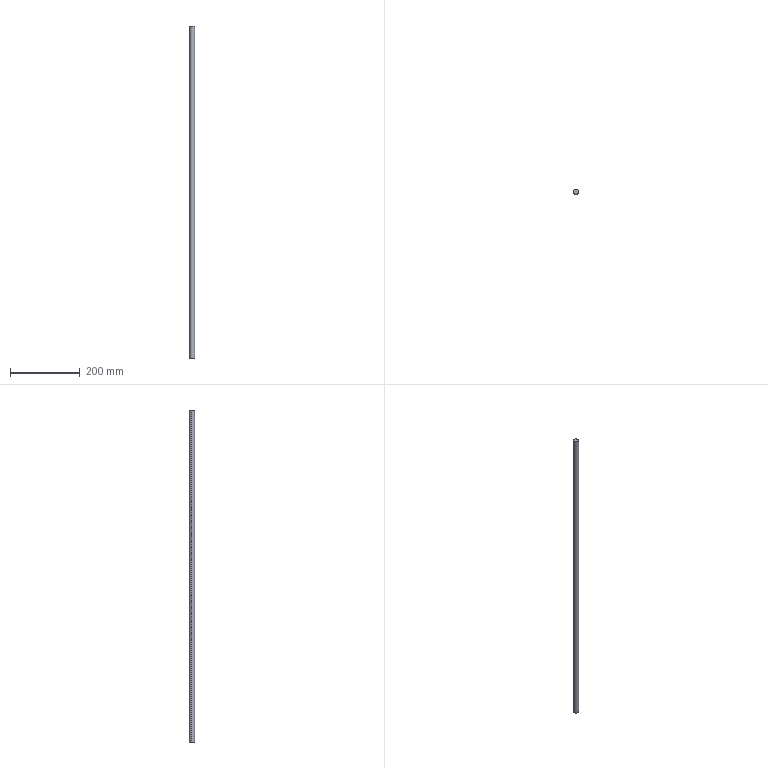Component | SolidWorks | ScrewRod1-2 | 1 solid | 4 faces | box 15 x 15 x 950 mm | volume 167879 mm3 | cylinder 2 | plane 2 | commonest cylinder face diameters 15 x2 | material 1023 Carbon Steel Plate (SS)
build123d program:
from build123d import *

# Parameters (mm, degrees)
SKETCH1_R           = 7.5
BOSS_EXTRUDE1_DEPTH = 950


with BuildPart() as part:
    # Sketch1 → Boss-Extrude1 (new body)
    with BuildSketch(Plane.XY):
        with Locations(Location((0, 0, 0), (0, 0, 180))):
            Circle(SKETCH1_R)
    extrude(amount=BOSS_EXTRUDE1_DEPTH)


solid = part.part

# Placed as in the assembly
solid = solid.moved(Location((32.544, 42.584, -394.606), (0, 0, 0)))
STEP:
#1=COLOUR_RGB('',0.7922,0.8196,0.9333);
#2=FILL_AREA_STYLE_COLOUR('',#1);
#3=FILL_AREA_STYLE('',(#2));
#4=SURFACE_STYLE_FILL_AREA(#3);
#5=SURFACE_SIDE_STYLE('',(#4));
#6=SURFACE_STYLE_USAGE(.BOTH.,#5);
#7=PRESENTATION_STYLE_ASSIGNMENT((#6));
#8=CARTESIAN_POINT('',(0.993,1.741,21.866));
#9=VERTEX_POINT('',#8);
#10=CARTESIAN_POINT('',(1.57,1.612,21.866));
#11=VERTEX_POINT('',#10);
#12=CARTESIAN_POINT('',(1.281,1.677,21.866));
#13=DIRECTION('',(0.,0.,1.));
#14=DIRECTION('',(-0.9762,0.217,0.));
#15=AXIS2_PLACEMENT_3D('',#12,#13,#14);
#16=CIRCLE('',#15,0.2953);
#17=EDGE_CURVE('',#9,#11,#16,.T.);
#18=ORIENTED_EDGE('',*,*,#17,.F.);
#19=CARTESIAN_POINT('',(0.993,1.741,-15.536));
#20=VERTEX_POINT('',#19);
#21=CARTESIAN_POINT('',(0.993,1.741,21.866));
#22=DIRECTION('',(0.,0.,-1.));
#23=VECTOR('',#22,39.37);
#24=LINE('',#21,#23);
#25=EDGE_CURVE('',#9,#20,#24,.T.);
#26=ORIENTED_EDGE('',*,*,#25,.T.);
#27=CARTESIAN_POINT('',(1.57,1.612,-15.536));
#28=VERTEX_POINT('',#27);
#29=CARTESIAN_POINT('',(1.281,1.677,-15.536));
#30=DIRECTION('',(0.,0.,1.));
#31=DIRECTION('',(-0.9762,0.217,0.));
#32=AXIS2_PLACEMENT_3D('',#29,#30,#31);
#33=CIRCLE('',#32,0.2953);
#34=EDGE_CURVE('',#20,#28,#33,.T.);
#35=ORIENTED_EDGE('',*,*,#34,.T.);
#36=CARTESIAN_POINT('',(1.57,1.612,21.866));
#37=DIRECTION('',(0.,0.,-1.));
#38=VECTOR('',#37,39.37);
#39=LINE('',#36,#38);
#40=EDGE_CURVE('',#11,#28,#39,.T.);
#41=ORIENTED_EDGE('',*,*,#40,.F.);
#42=EDGE_LOOP('',(#18,#26,#35,#41));
#43=FACE_OUTER_BOUND('',#42,.T.);
#44=CARTESIAN_POINT('',(1.281,1.677,21.866));
#45=DIRECTION('',(0.,0.,-1.));
#46=DIRECTION('',(0.9762,-0.217,0.));
#47=AXIS2_PLACEMENT_3D('',#44,#45,#46);
#48=CYLINDRICAL_SURFACE('',#47,0.2953);
#49=ADVANCED_FACE('',(#43),#48,.T.);
#50=ORIENTED_EDGE('',*,*,#25,.F.);
#51=CARTESIAN_POINT('',(1.281,1.677,21.866));
#52=DIRECTION('',(0.,0.,1.));
#53=DIRECTION('',(-0.9762,0.217,0.));
#54=AXIS2_PLACEMENT_3D('',#51,#52,#53);
#55=CIRCLE('',#54,0.2953);
#56=EDGE_CURVE('',#11,#9,#55,.T.);
#57=ORIENTED_EDGE('',*,*,#56,.F.);
#58=ORIENTED_EDGE('',*,*,#40,.T.);
#59=CARTESIAN_POINT('',(1.281,1.677,-15.536));
#60=DIRECTION('',(0.,0.,1.));
#61=DIRECTION('',(-0.9762,0.217,0.));
#62=AXIS2_PLACEMENT_3D('',#59,#60,#61);
#63=CIRCLE('',#62,0.2953);
#64=EDGE_CURVE('',#28,#20,#63,.T.);
#65=ORIENTED_EDGE('',*,*,#64,.T.);
#66=EDGE_LOOP('',(#50,#57,#58,#65));
#67=FACE_OUTER_BOUND('',#66,.T.);
#68=CARTESIAN_POINT('',(1.281,1.677,21.866));
#69=DIRECTION('',(0.,0.,-1.));
#70=DIRECTION('',(0.9762,-0.217,0.));
#71=AXIS2_PLACEMENT_3D('',#68,#69,#70);
#72=CYLINDRICAL_SURFACE('',#71,0.2953);
#73=ADVANCED_FACE('',(#67),#72,.T.);
#74=ORIENTED_EDGE('',*,*,#56,.T.);
#75=ORIENTED_EDGE('',*,*,#17,.T.);
#76=EDGE_LOOP('',(#74,#75));
#77=FACE_OUTER_BOUND('',#76,.T.);
#78=CARTESIAN_POINT('',(1.281,1.677,21.866));
#79=DIRECTION('',(0.,0.,1.));
#80=DIRECTION('',(-0.9762,0.217,0.));
#81=AXIS2_PLACEMENT_3D('',#78,#79,#80);
#82=PLANE('',#81);
#83=ADVANCED_FACE('',(#77),#82,.T.);
#84=ORIENTED_EDGE('',*,*,#64,.F.);
#85=ORIENTED_EDGE('',*,*,#34,.F.);
#86=EDGE_LOOP('',(#84,#85));
#87=FACE_OUTER_BOUND('',#86,.T.);
#88=CARTESIAN_POINT('',(1.281,1.677,-15.536));
#89=DIRECTION('',(0.,0.,1.));
#90=DIRECTION('',(-0.9762,0.217,0.));
#91=AXIS2_PLACEMENT_3D('',#88,#89,#90);
#92=PLANE('',#91);
#93=ADVANCED_FACE('',(#87),#92,.F.);
#94=CLOSED_SHELL('',(#49,#73,#83,#93));
#95=MANIFOLD_SOLID_BREP('',#94);
#96=STYLED_ITEM('',(#7),#95);
#97=(LENGTH_UNIT()NAMED_UNIT(*)SI_UNIT($,.METRE.));
#98=LENGTH_MEASURE_WITH_UNIT(LENGTH_MEASURE(0.0254),#97);
#99=DIMENSIONAL_EXPONENTS(1.,0.,0.,0.,0.,0.,0.);
#100=(CONVERSION_BASED_UNIT('',#98)LENGTH_UNIT()NAMED_UNIT(#99));
#101=UNCERTAINTY_MEASURE_WITH_UNIT(LENGTH_MEASURE(0.00001),#100,'','');
#102=(NAMED_UNIT(*)PLANE_ANGLE_UNIT()SI_UNIT($,.RADIAN.));
#103=(NAMED_UNIT(*)SI_UNIT($,.STERADIAN.)SOLID_ANGLE_UNIT());
#104=(GEOMETRIC_REPRESENTATION_CONTEXT(3)GLOBAL_UNCERTAINTY_ASSIGNED_CONTEXT((#101))GLOBAL_UNIT_ASSIGNED_CONTEXT((#100,#102,#103))REPRESENTATION_CONTEXT('',''));
#105=MECHANICAL_DESIGN_GEOMETRIC_PRESENTATION_REPRESENTATION('',(#96),#104);
#106=PRESENTATION_LAYER_ASSIGNMENT('','',(#96));
#107=CARTESIAN_POINT('',(0.,0.,0.));
#108=DIRECTION('',(0.,0.,1.));
#109=DIRECTION('',(1.,0.,0.));
#110=AXIS2_PLACEMENT_3D('',#107,#108,#109);
#111=(LENGTH_UNIT()NAMED_UNIT(*)SI_UNIT($,.METRE.));
#112=LENGTH_MEASURE_WITH_UNIT(LENGTH_MEASURE(0.0254),#111);
#113=DIMENSIONAL_EXPONENTS(1.,0.,0.,0.,0.,0.,0.);
#114=(CONVERSION_BASED_UNIT('',#112)LENGTH_UNIT()NAMED_UNIT(#113));
#115=UNCERTAINTY_MEASURE_WITH_UNIT(LENGTH_MEASURE(0.00001),#114,'','');
#116=(NAMED_UNIT(*)PLANE_ANGLE_UNIT()SI_UNIT($,.RADIAN.));
#117=(NAMED_UNIT(*)SI_UNIT($,.STERADIAN.)SOLID_ANGLE_UNIT());
#118=(GEOMETRIC_REPRESENTATION_CONTEXT(3)GLOBAL_UNCERTAINTY_ASSIGNED_CONTEXT((#115))GLOBAL_UNIT_ASSIGNED_CONTEXT((#114,#116,#117))REPRESENTATION_CONTEXT('',''));
#119=ADVANCED_BREP_SHAPE_REPRESENTATION('',(#95,#110),#118);